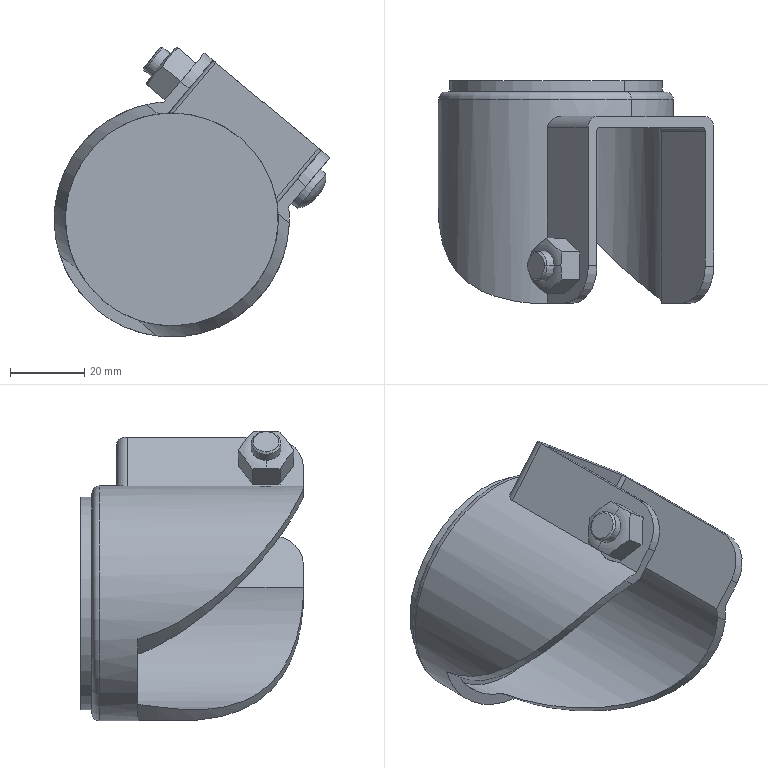Component | SolidWorks | 30-01A-1_Wheel-322-1_CJH65-322-1_CJH65body-322-1 | 1 solid | 48 faces | box 74.19 x 59.9 x 78.07 mm | volume 49149 mm3 | cylinder 20 | plane 20 | torus 6 | cone 2 | commonest cylinder face diameters 57.333 x4 8 x2 16 x2 12 x2 63.333 x2 6 x2 20 x2 104 x2
build123d program:
from build123d import *

# Parameters (mm, degrees)
EXTRUDE1_DEPTH          = 90
CUT_EXTRUDE1_DEPTH      = 90
CUT_EXTRUDE2_START      = -92
SKETCH4_R               = 28.667
CUT_EXTRUDE2_DEPTH      = 92
CUT_EXTRUDE3_DEPTH      = 92
CUT_EXTRUDE3_DEPTH_BACK = 92
SKETCH8_R               = 8
CUT_EXTRUDE4_DEPTH      = 92


with BuildPart() as part:
    # Sketch1 → Revolve1 (revolve)
    with BuildSketch(Plane.XY, mode=Mode.PRIVATE) as revolve1_sk:
        with BuildLine():
            Line((0, -9.6), (28.667, -9.6))
            Line((28.667, -9.6), (28.667, -12.6))
            Line((28.667, -12.6), (29.667, -12.6))
            ThreePointArc((29.667, -12.6), (31.081, -13.186), (31.667, -14.6))
            Line((31.667, -14.6), (31.667, -88.8))
            Line((31.667, -88.8), (0, -88.8))
            Line((0, -88.8), (0, -9.6))
        make_face()
    revolve(revolve1_sk.sketch.rotate(Axis((0, -88.8, 0), (0, 1, 0)), 270), axis=Axis((0, -88.8, 0), (0, 1, 0)))

    # Sketch2 → Extrude1 (add)
    with BuildSketch(Plane.XY):
        with BuildLine():
            Line((-22, -85.6), (22, -85.6))
            Line((22, -85.6), (22, -22.2))
            ThreePointArc((22, -22.2), (21.121, -20.079), (19, -19.2))
            Line((19, -19.2), (-19, -19.2))
            ThreePointArc((-19, -19.2), (-21.121, -20.079), (-22, -22.2))
            Line((-22, -22.2), (-22, -85.6))
        make_face()
    extrude(amount=EXTRUDE1_DEPTH)

    # Sketch3 → Cut-Extrude1 (cut)
    with BuildSketch(Plane.XY):
        with BuildLine():
            Line((-19, -85.6), (19, -85.6))
            Line((19, -85.6), (19, -23.2))
            ThreePointArc((19, -23.2), (18.707, -22.493), (18, -22.2))
            Line((18, -22.2), (-18, -22.2))
            ThreePointArc((-18, -22.2), (-18.707, -22.493), (-19, -23.2))
            Line((-19, -23.2), (-19, -85.6))
        make_face()
    extrude(amount=CUT_EXTRUDE1_DEPTH, mode=Mode.SUBTRACT)

    # Sketch4 → Cut-Extrude2 (cut)
    with BuildSketch(Plane(origin=(0, -18.8, 0), x_dir=(-1, 0, 0), z_dir=(0, 1, 0)).offset(CUT_EXTRUDE2_START)):
        with Locations(Location((0, 0, 0), (0, 0, 90))):
            Circle(SKETCH4_R)
    extrude(amount=CUT_EXTRUDE2_DEPTH, mode=Mode.SUBTRACT)

    # Sketch5 → Cut-Extrude3 (cut, two sides: drawn at the far end of the back side and taken through both)
    with BuildSketch(Plane(origin=(0, 0, 0), x_dir=(0, 0, -1), z_dir=(1, 0, 0)).offset(-CUT_EXTRUDE3_DEPTH_BACK)):
        with BuildLine():
            Line((-200, 0), (-200, -200))
            Line((-200, -200), (200, -200))
            Line((200, -200), (200, 0))
            Line((200, 0), (50, 0))
            Line((50, 0), (50, -25))
            Line((50, -25), (26.667, -25))
            ThreePointArc((26.667, -25), (11.284, -55.195), (-19.437, -69.5))
            Line((-19.437, -69.5), (-30, -69.5))
            ThreePointArc((-30, -69.5), (-37.071, -66.571), (-40, -59.5))
            Line((-40, -59.5), (-40, 0))
            Line((-40, 0), (-200, 0))
        make_face()
    extrude(amount=CUT_EXTRUDE3_DEPTH + CUT_EXTRUDE3_DEPTH_BACK, mode=Mode.SUBTRACT)

    # Sketch6 → Rotate2 (revolve)
    with BuildSketch(Plane.XY.offset(30), mode=Mode.PRIVATE) as rotate2_sk:
        with BuildLine():
            Line((22, -59.5), (22, -53.5))
            Line((22, -53.5), (24, -53.5))
            ThreePointArc((24, -53.5), (25.716, -56.261), (26, -59.5))
            Line((26, -59.5), (22, -59.5))
        make_face()
    revolve(rotate2_sk.sketch.rotate(Axis((26, -59.5, 30), (-1, 0, 0)), 270), axis=Axis((26, -59.5, 30), (-1, 0, 0)))

    # Sketch7 → Rotate3 (revolve)
    with BuildSketch(Plane.XY.offset(30), mode=Mode.PRIVATE) as rotate3_sk:
        with BuildLine():
            Line((-32, -59.5), (-32, -56))
            Line((-32, -56), (-31.5, -55.5))
            Line((-31.5, -55.5), (-29, -55.5))
            ThreePointArc((-29, -55.5), (-28.801, -53.425), (-28, -51.5))
            Line((-28, -51.5), (-22, -51.5))
            Line((-22, -51.5), (-22, -59.5))
            Line((-22, -59.5), (-32, -59.5))
        make_face()
    revolve(rotate3_sk.sketch.rotate(Axis((-22, -59.5, 30), (-1, 0, 0)), 270), axis=Axis((-22, -59.5, 30), (-1, 0, 0)))

    # Sketch8 → Cut-Extrude4 (cut)
    with BuildSketch(Plane(origin=(-22, 0, 0), x_dir=(0, 0, -1), z_dir=(1, 0, 0))):
        with Locations((-30, -59.5)):
            Circle(SKETCH8_R)
        Polygon((-36.5, -55.747), (-36.5, -63.253), (-30, -67.006), (-23.5, -63.253), (-23.5, -55.747), (-30, -51.994), align=None, mode=Mode.SUBTRACT)
    extrude(amount=-CUT_EXTRUDE4_DEPTH, mode=Mode.SUBTRACT)


solid = part.part

# Placed as in the assembly
solid = solid.moved(Location((158.07, -562.845, -114.5), (-0.0002872, 39.864, 0)))